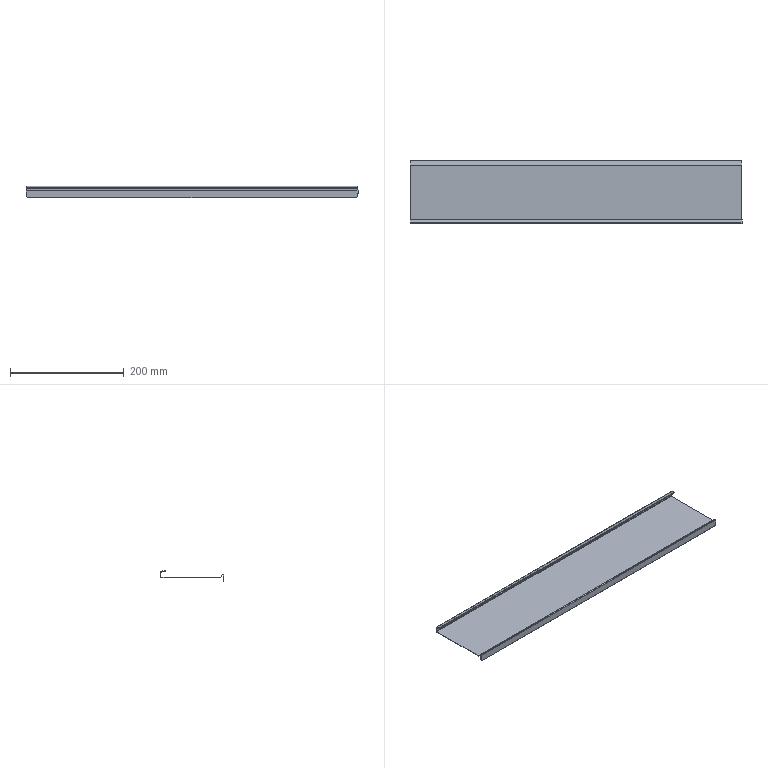Component | SolidWorks | PC-CAJ-P08-1_PC-CAJ-P17-2_PM-CAJ-P54-1 | 1 solid | 50 faces | volume 62127 mm3 | plane 38 | cylinder 12 | commonest cylinder face diameters 2.4 x5 1 x4 0.2 x2 1.6 x1 | material Plain Carbon Steel